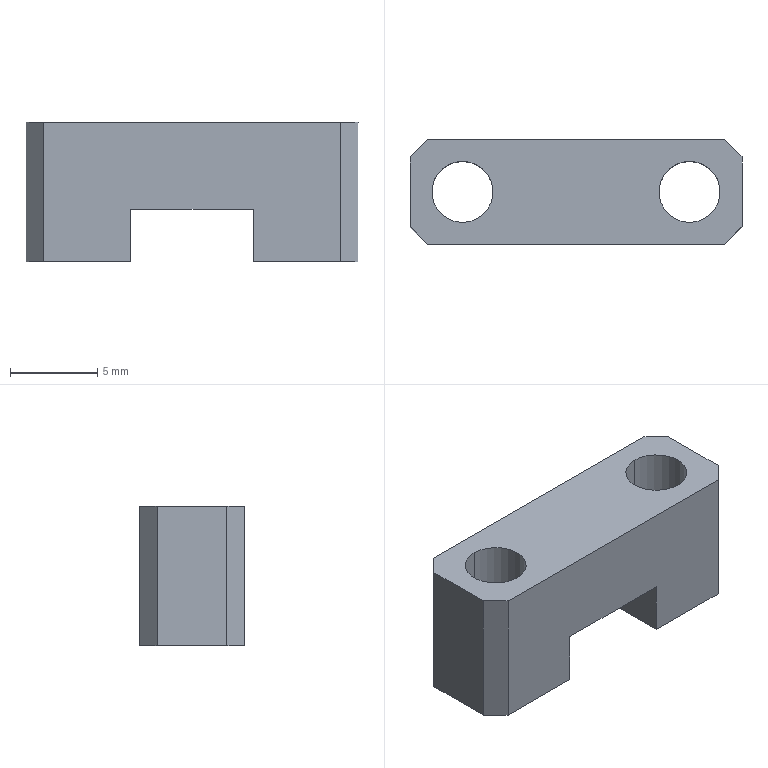Component | SolidWorks | F01AE00111-A5175-1 | 1 solid | 18 faces | box 19 x 6 x 8 mm | volume 616 mm3 | plane 14 | cylinder 4 | commonest cylinder face diameters 3.5 x4 | material 6061 Alloy
build123d program:
from build123d import *

# Parameters (mm, degrees)
BOSS_EXTRUDE1_DEPTH        = 3
F_3_5_3_5_DIAMETER_HOLE1_D = 3.5
CHAMFER1_SIZE              = 1


with BuildPart() as part:
    # Sketch1 → Boss-Extrude1 (new, symmetric)
    with BuildSketch(Plane.XY):
        Polygon((3.5, 0), (-3.5, 0), (-3.5, 3), (-9.5, 3), (-9.5, -5), (9.5, -5), (9.5, 3), (3.5, 3), align=None)
    extrude(amount=BOSS_EXTRUDE1_DEPTH, both=True)

    # 3.5 _3.5_ Diameter Hole1 (through all)
    with Locations(Plane(origin=(0, -5, 0), x_dir=(-1, 0, 0), z_dir=(0, -1, 0))):
        with Locations((-6.5, 0), (6.5, 0)):
            Hole(F_3_5_3_5_DIAMETER_HOLE1_D / 2)

    # Chamfer1
    chamfer1_edges = [part.edges().sort_by_distance(p)[0] for p in [
        (-9.5, -1, 3),
        (9.5, -1, 3),
        (9.5, -1, -3),
        (-9.5, -1, -3),
    ]]
    chamfer(chamfer1_edges, length=CHAMFER1_SIZE)


solid = part.part

# Placed as in the assembly
solid = solid.moved(Location((-63.681, -106.773, -304.179), (-90, 0, 0)))
STEP:
#1=CARTESIAN_POINT('',(-2.251,-4.135,-12.094));
#2=VERTEX_POINT('',#1);
#3=CARTESIAN_POINT('',(-2.251,-4.273,-12.094));
#4=VERTEX_POINT('',#3);
#5=CARTESIAN_POINT('',(-2.251,-4.204,-12.094));
#6=DIRECTION('',(0.,-0.,1.));
#7=DIRECTION('',(0.,-1.,0.));
#8=AXIS2_PLACEMENT_3D('',#5,#6,#7);
#9=CIRCLE('',#8,0.0689);
#10=EDGE_CURVE('',#2,#4,#9,.T.);
#11=ORIENTED_EDGE('',*,*,#10,.F.);
#12=CARTESIAN_POINT('',(-2.251,-4.135,-11.779));
#13=VERTEX_POINT('',#12);
#14=CARTESIAN_POINT('',(-2.251,-4.135,-11.779));
#15=DIRECTION('',(0.,-0.,1.));
#16=VECTOR('',#15,39.37);
#17=LINE('',#14,#16);
#18=EDGE_CURVE('',#2,#13,#17,.T.);
#19=ORIENTED_EDGE('',*,*,#18,.T.);
#20=CARTESIAN_POINT('',(-2.251,-4.273,-11.779));
#21=VERTEX_POINT('',#20);
#22=CARTESIAN_POINT('',(-2.251,-4.204,-11.779));
#23=DIRECTION('',(0.,-0.,1.));
#24=DIRECTION('',(0.,-1.,0.));
#25=AXIS2_PLACEMENT_3D('',#22,#23,#24);
#26=CIRCLE('',#25,0.0689);
#27=EDGE_CURVE('',#13,#21,#26,.T.);
#28=ORIENTED_EDGE('',*,*,#27,.T.);
#29=CARTESIAN_POINT('',(-2.251,-4.273,-11.779));
#30=DIRECTION('',(0.,-0.,1.));
#31=VECTOR('',#30,39.37);
#32=LINE('',#29,#31);
#33=EDGE_CURVE('',#4,#21,#32,.T.);
#34=ORIENTED_EDGE('',*,*,#33,.F.);
#35=EDGE_LOOP('',(#11,#19,#28,#34));
#36=FACE_OUTER_BOUND('',#35,.T.);
#37=CARTESIAN_POINT('',(-2.251,-4.204,-11.779));
#38=DIRECTION('',(0.,-0.,1.));
#39=DIRECTION('',(0.,-1.,0.));
#40=AXIS2_PLACEMENT_3D('',#37,#38,#39);
#41=CYLINDRICAL_SURFACE('',#40,0.0689);
#42=ADVANCED_FACE('',(#36),#41,.F.);
#43=CARTESIAN_POINT('',(-2.763,-4.135,-12.094));
#44=VERTEX_POINT('',#43);
#45=CARTESIAN_POINT('',(-2.763,-4.273,-12.094));
#46=VERTEX_POINT('',#45);
#47=CARTESIAN_POINT('',(-2.763,-4.204,-12.094));
#48=DIRECTION('',(0.,-0.,1.));
#49=DIRECTION('',(0.,-1.,0.));
#50=AXIS2_PLACEMENT_3D('',#47,#48,#49);
#51=CIRCLE('',#50,0.0689);
#52=EDGE_CURVE('',#44,#46,#51,.T.);
#53=ORIENTED_EDGE('',*,*,#52,.F.);
#54=CARTESIAN_POINT('',(-2.763,-4.135,-11.779));
#55=VERTEX_POINT('',#54);
#56=CARTESIAN_POINT('',(-2.763,-4.135,-11.779));
#57=DIRECTION('',(0.,-0.,1.));
#58=VECTOR('',#57,39.37);
#59=LINE('',#56,#58);
#60=EDGE_CURVE('',#44,#55,#59,.T.);
#61=ORIENTED_EDGE('',*,*,#60,.T.);
#62=CARTESIAN_POINT('',(-2.763,-4.273,-11.779));
#63=VERTEX_POINT('',#62);
#64=CARTESIAN_POINT('',(-2.763,-4.204,-11.779));
#65=DIRECTION('',(0.,-0.,1.));
#66=DIRECTION('',(0.,-1.,0.));
#67=AXIS2_PLACEMENT_3D('',#64,#65,#66);
#68=CIRCLE('',#67,0.0689);
#69=EDGE_CURVE('',#55,#63,#68,.T.);
#70=ORIENTED_EDGE('',*,*,#69,.T.);
#71=CARTESIAN_POINT('',(-2.763,-4.273,-11.779));
#72=DIRECTION('',(0.,-0.,1.));
#73=VECTOR('',#72,39.37);
#74=LINE('',#71,#73);
#75=EDGE_CURVE('',#46,#63,#74,.T.);
#76=ORIENTED_EDGE('',*,*,#75,.F.);
#77=EDGE_LOOP('',(#53,#61,#70,#76));
#78=FACE_OUTER_BOUND('',#77,.T.);
#79=CARTESIAN_POINT('',(-2.763,-4.204,-11.779));
#80=DIRECTION('',(0.,-0.,1.));
#81=DIRECTION('',(0.,-1.,0.));
#82=AXIS2_PLACEMENT_3D('',#79,#80,#81);
#83=CYLINDRICAL_SURFACE('',#82,0.0689);
#84=ADVANCED_FACE('',(#78),#83,.F.);
#85=CARTESIAN_POINT('',(-2.645,-4.322,-11.976));
#86=VERTEX_POINT('',#85);
#87=CARTESIAN_POINT('',(-2.645,-4.322,-12.094));
#88=VERTEX_POINT('',#87);
#89=CARTESIAN_POINT('',(-2.645,-4.322,-11.976));
#90=DIRECTION('',(-0.,0.,-1.));
#91=VECTOR('',#90,39.37);
#92=LINE('',#89,#91);
#93=EDGE_CURVE('',#86,#88,#92,.T.);
#94=ORIENTED_EDGE('',*,*,#93,.T.);
#95=CARTESIAN_POINT('',(-2.645,-4.086,-12.094));
#96=VERTEX_POINT('',#95);
#97=CARTESIAN_POINT('',(-2.645,-4.086,-12.094));
#98=DIRECTION('',(-0.,-1.,-0.));
#99=VECTOR('',#98,39.37);
#100=LINE('',#97,#99);
#101=EDGE_CURVE('',#96,#88,#100,.T.);
#102=ORIENTED_EDGE('',*,*,#101,.F.);
#103=CARTESIAN_POINT('',(-2.645,-4.086,-11.976));
#104=VERTEX_POINT('',#103);
#105=CARTESIAN_POINT('',(-2.645,-4.086,-11.976));
#106=DIRECTION('',(-0.,0.,-1.));
#107=VECTOR('',#106,39.37);
#108=LINE('',#105,#107);
#109=EDGE_CURVE('',#104,#96,#108,.T.);
#110=ORIENTED_EDGE('',*,*,#109,.F.);
#111=CARTESIAN_POINT('',(-2.645,-4.086,-11.976));
#112=DIRECTION('',(-0.,-1.,-0.));
#113=VECTOR('',#112,39.37);
#114=LINE('',#111,#113);
#115=EDGE_CURVE('',#104,#86,#114,.T.);
#116=ORIENTED_EDGE('',*,*,#115,.T.);
#117=EDGE_LOOP('',(#94,#102,#110,#116));
#118=FACE_OUTER_BOUND('',#117,.T.);
#119=CARTESIAN_POINT('',(-2.645,-4.086,-11.976));
#120=DIRECTION('',(-1.,0.,0.));
#121=DIRECTION('',(0.,1.,0.));
#122=AXIS2_PLACEMENT_3D('',#119,#120,#121);
#123=PLANE('',#122);
#124=ADVANCED_FACE('',(#118),#123,.F.);
#125=CARTESIAN_POINT('',(-2.763,-4.204,-12.094));
#126=DIRECTION('',(0.,-0.,1.));
#127=DIRECTION('',(0.,-1.,0.));
#128=AXIS2_PLACEMENT_3D('',#125,#126,#127);
#129=CIRCLE('',#128,0.0689);
#130=EDGE_CURVE('',#46,#44,#129,.T.);
#131=ORIENTED_EDGE('',*,*,#130,.T.);
#132=ORIENTED_EDGE('',*,*,#52,.T.);
#133=EDGE_LOOP('',(#131,#132));
#134=FACE_BOUND('',#133,.T.);
#135=CARTESIAN_POINT('',(-2.842,-4.322,-12.094));
#136=VERTEX_POINT('',#135);
#137=CARTESIAN_POINT('',(-2.645,-4.322,-12.094));
#138=DIRECTION('',(-1.,0.,0.));
#139=VECTOR('',#138,39.37);
#140=LINE('',#137,#139);
#141=EDGE_CURVE('',#88,#136,#140,.T.);
#142=ORIENTED_EDGE('',*,*,#141,.T.);
#143=CARTESIAN_POINT('',(-2.881,-4.282,-12.094));
#144=VERTEX_POINT('',#143);
#145=CARTESIAN_POINT('',(-2.881,-4.282,-12.094));
#146=DIRECTION('',(-0.7071,0.7071,0.));
#147=VECTOR('',#146,39.37);
#148=LINE('',#145,#147);
#149=EDGE_CURVE('',#136,#144,#148,.T.);
#150=ORIENTED_EDGE('',*,*,#149,.T.);
#151=CARTESIAN_POINT('',(-2.881,-4.125,-12.094));
#152=VERTEX_POINT('',#151);
#153=CARTESIAN_POINT('',(-2.881,-4.086,-12.094));
#154=DIRECTION('',(-0.,-1.,-0.));
#155=VECTOR('',#154,39.37);
#156=LINE('',#153,#155);
#157=EDGE_CURVE('',#152,#144,#156,.T.);
#158=ORIENTED_EDGE('',*,*,#157,.F.);
#159=CARTESIAN_POINT('',(-2.842,-4.086,-12.094));
#160=VERTEX_POINT('',#159);
#161=CARTESIAN_POINT('',(-2.842,-4.086,-12.094));
#162=DIRECTION('',(0.7071,0.7071,-0.));
#163=VECTOR('',#162,39.37);
#164=LINE('',#161,#163);
#165=EDGE_CURVE('',#152,#160,#164,.T.);
#166=ORIENTED_EDGE('',*,*,#165,.T.);
#167=CARTESIAN_POINT('',(-2.645,-4.086,-12.094));
#168=DIRECTION('',(-1.,0.,0.));
#169=VECTOR('',#168,39.37);
#170=LINE('',#167,#169);
#171=EDGE_CURVE('',#96,#160,#170,.T.);
#172=ORIENTED_EDGE('',*,*,#171,.F.);
#173=ORIENTED_EDGE('',*,*,#101,.T.);
#174=EDGE_LOOP('',(#142,#150,#158,#166,#172,#173));
#175=FACE_OUTER_BOUND('',#174,.T.);
#176=CARTESIAN_POINT('',(-2.645,-4.086,-12.094));
#177=DIRECTION('',(0.,-0.,1.));
#178=DIRECTION('',(-0.,-1.,-0.));
#179=AXIS2_PLACEMENT_3D('',#176,#177,#178);
#180=PLANE('',#179);
#181=ADVANCED_FACE('',(#134,#175),#180,.F.);
#182=ORIENTED_EDGE('',*,*,#157,.T.);
#183=CARTESIAN_POINT('',(-2.881,-4.282,-11.779));
#184=VERTEX_POINT('',#183);
#185=CARTESIAN_POINT('',(-2.881,-4.282,-12.094));
#186=DIRECTION('',(0.,-0.,1.));
#187=VECTOR('',#186,39.37);
#188=LINE('',#185,#187);
#189=EDGE_CURVE('',#144,#184,#188,.T.);
#190=ORIENTED_EDGE('',*,*,#189,.T.);
#191=CARTESIAN_POINT('',(-2.881,-4.125,-11.779));
#192=VERTEX_POINT('',#191);
#193=CARTESIAN_POINT('',(-2.881,-4.086,-11.779));
#194=DIRECTION('',(-0.,-1.,-0.));
#195=VECTOR('',#194,39.37);
#196=LINE('',#193,#195);
#197=EDGE_CURVE('',#192,#184,#196,.T.);
#198=ORIENTED_EDGE('',*,*,#197,.F.);
#199=CARTESIAN_POINT('',(-2.881,-4.125,-12.094));
#200=DIRECTION('',(-0.,0.,-1.));
#201=VECTOR('',#200,39.37);
#202=LINE('',#199,#201);
#203=EDGE_CURVE('',#192,#152,#202,.T.);
#204=ORIENTED_EDGE('',*,*,#203,.T.);
#205=EDGE_LOOP('',(#182,#190,#198,#204));
#206=FACE_OUTER_BOUND('',#205,.T.);
#207=CARTESIAN_POINT('',(-2.881,-4.086,-12.094));
#208=DIRECTION('',(1.,-0.,-0.));
#209=DIRECTION('',(-0.,0.,-1.));
#210=AXIS2_PLACEMENT_3D('',#207,#208,#209);
#211=PLANE('',#210);
#212=ADVANCED_FACE('',(#206),#211,.F.);
#213=CARTESIAN_POINT('',(-2.251,-4.204,-11.779));
#214=DIRECTION('',(0.,-0.,1.));
#215=DIRECTION('',(0.,-1.,0.));
#216=AXIS2_PLACEMENT_3D('',#213,#214,#215);
#217=CIRCLE('',#216,0.0689);
#218=EDGE_CURVE('',#21,#13,#217,.T.);
#219=ORIENTED_EDGE('',*,*,#218,.F.);
#220=ORIENTED_EDGE('',*,*,#27,.F.);
#221=EDGE_LOOP('',(#219,#220));
#222=FACE_BOUND('',#221,.T.);
#223=CARTESIAN_POINT('',(-2.763,-4.204,-11.779));
#224=DIRECTION('',(0.,-0.,1.));
#225=DIRECTION('',(0.,-1.,0.));
#226=AXIS2_PLACEMENT_3D('',#223,#224,#225);
#227=CIRCLE('',#226,0.0689);
#228=EDGE_CURVE('',#63,#55,#227,.T.);
#229=ORIENTED_EDGE('',*,*,#228,.F.);
#230=ORIENTED_EDGE('',*,*,#69,.F.);
#231=EDGE_LOOP('',(#229,#230));
#232=FACE_BOUND('',#231,.T.);
#233=CARTESIAN_POINT('',(-2.842,-4.322,-11.779));
#234=VERTEX_POINT('',#233);
#235=CARTESIAN_POINT('',(-2.172,-4.322,-11.779));
#236=VERTEX_POINT('',#235);
#237=CARTESIAN_POINT('',(-2.881,-4.322,-11.779));
#238=DIRECTION('',(1.,-0.,-0.));
#239=VECTOR('',#238,39.37);
#240=LINE('',#237,#239);
#241=EDGE_CURVE('',#234,#236,#240,.T.);
#242=ORIENTED_EDGE('',*,*,#241,.T.);
#243=CARTESIAN_POINT('',(-2.133,-4.282,-11.779));
#244=VERTEX_POINT('',#243);
#245=CARTESIAN_POINT('',(-2.133,-4.282,-11.779));
#246=DIRECTION('',(0.7071,0.7071,-0.));
#247=VECTOR('',#246,39.37);
#248=LINE('',#245,#247);
#249=EDGE_CURVE('',#236,#244,#248,.T.);
#250=ORIENTED_EDGE('',*,*,#249,.T.);
#251=CARTESIAN_POINT('',(-2.133,-4.125,-11.779));
#252=VERTEX_POINT('',#251);
#253=CARTESIAN_POINT('',(-2.133,-4.086,-11.779));
#254=DIRECTION('',(-0.,-1.,-0.));
#255=VECTOR('',#254,39.37);
#256=LINE('',#253,#255);
#257=EDGE_CURVE('',#252,#244,#256,.T.);
#258=ORIENTED_EDGE('',*,*,#257,.F.);
#259=CARTESIAN_POINT('',(-2.172,-4.086,-11.779));
#260=VERTEX_POINT('',#259);
#261=CARTESIAN_POINT('',(-2.172,-4.086,-11.779));
#262=DIRECTION('',(-0.7071,0.7071,0.));
#263=VECTOR('',#262,39.37);
#264=LINE('',#261,#263);
#265=EDGE_CURVE('',#252,#260,#264,.T.);
#266=ORIENTED_EDGE('',*,*,#265,.T.);
#267=CARTESIAN_POINT('',(-2.842,-4.086,-11.779));
#268=VERTEX_POINT('',#267);
#269=CARTESIAN_POINT('',(-2.881,-4.086,-11.779));
#270=DIRECTION('',(1.,-0.,-0.));
#271=VECTOR('',#270,39.37);
#272=LINE('',#269,#271);
#273=EDGE_CURVE('',#268,#260,#272,.T.);
#274=ORIENTED_EDGE('',*,*,#273,.F.);
#275=CARTESIAN_POINT('',(-2.842,-4.086,-11.779));
#276=DIRECTION('',(-0.7071,-0.7071,0.));
#277=VECTOR('',#276,39.37);
#278=LINE('',#275,#277);
#279=EDGE_CURVE('',#268,#192,#278,.T.);
#280=ORIENTED_EDGE('',*,*,#279,.T.);
#281=ORIENTED_EDGE('',*,*,#197,.T.);
#282=CARTESIAN_POINT('',(-2.881,-4.282,-11.779));
#283=DIRECTION('',(0.7071,-0.7071,-0.));
#284=VECTOR('',#283,39.37);
#285=LINE('',#282,#284);
#286=EDGE_CURVE('',#184,#234,#285,.T.);
#287=ORIENTED_EDGE('',*,*,#286,.T.);
#288=EDGE_LOOP('',(#242,#250,#258,#266,#274,#280,#281,#287));
#289=FACE_OUTER_BOUND('',#288,.T.);
#290=CARTESIAN_POINT('',(-2.881,-4.086,-11.779));
#291=DIRECTION('',(-0.,0.,-1.));
#292=DIRECTION('',(-1.,0.,0.));
#293=AXIS2_PLACEMENT_3D('',#290,#291,#292);
#294=PLANE('',#293);
#295=ADVANCED_FACE('',(#222,#232,#289),#294,.F.);
#296=ORIENTED_EDGE('',*,*,#257,.T.);
#297=CARTESIAN_POINT('',(-2.133,-4.282,-12.094));
#298=VERTEX_POINT('',#297);
#299=CARTESIAN_POINT('',(-2.133,-4.282,-12.094));
#300=DIRECTION('',(-0.,0.,-1.));
#301=VECTOR('',#300,39.37);
#302=LINE('',#299,#301);
#303=EDGE_CURVE('',#244,#298,#302,.T.);
#304=ORIENTED_EDGE('',*,*,#303,.T.);
#305=CARTESIAN_POINT('',(-2.133,-4.125,-12.094));
#306=VERTEX_POINT('',#305);
#307=CARTESIAN_POINT('',(-2.133,-4.086,-12.094));
#308=DIRECTION('',(-0.,-1.,-0.));
#309=VECTOR('',#308,39.37);
#310=LINE('',#307,#309);
#311=EDGE_CURVE('',#306,#298,#310,.T.);
#312=ORIENTED_EDGE('',*,*,#311,.F.);
#313=CARTESIAN_POINT('',(-2.133,-4.125,-11.779));
#314=DIRECTION('',(0.,-0.,1.));
#315=VECTOR('',#314,39.37);
#316=LINE('',#313,#315);
#317=EDGE_CURVE('',#306,#252,#316,.T.);
#318=ORIENTED_EDGE('',*,*,#317,.T.);
#319=EDGE_LOOP('',(#296,#304,#312,#318));
#320=FACE_OUTER_BOUND('',#319,.T.);
#321=CARTESIAN_POINT('',(-2.133,-4.086,-12.094));
#322=DIRECTION('',(-1.,0.,0.));
#323=DIRECTION('',(0.,-0.,1.));
#324=AXIS2_PLACEMENT_3D('',#321,#322,#323);
#325=PLANE('',#324);
#326=ADVANCED_FACE('',(#320),#325,.F.);
#327=CARTESIAN_POINT('',(-2.251,-4.204,-12.094));
#328=DIRECTION('',(0.,-0.,1.));
#329=DIRECTION('',(0.,-1.,0.));
#330=AXIS2_PLACEMENT_3D('',#327,#328,#329);
#331=CIRCLE('',#330,0.0689);
#332=EDGE_CURVE('',#4,#2,#331,.T.);
#333=ORIENTED_EDGE('',*,*,#332,.T.);
#334=ORIENTED_EDGE('',*,*,#10,.T.);
#335=EDGE_LOOP('',(#333,#334));
#336=FACE_BOUND('',#335,.T.);
#337=ORIENTED_EDGE('',*,*,#311,.T.);
#338=CARTESIAN_POINT('',(-2.172,-4.322,-12.094));
#339=VERTEX_POINT('',#338);
#340=CARTESIAN_POINT('',(-2.133,-4.282,-12.094));
#341=DIRECTION('',(-0.7071,-0.7071,0.));
#342=VECTOR('',#341,39.37);
#343=LINE('',#340,#342);
#344=EDGE_CURVE('',#298,#339,#343,.T.);
#345=ORIENTED_EDGE('',*,*,#344,.T.);
#346=CARTESIAN_POINT('',(-2.369,-4.322,-12.094));
#347=VERTEX_POINT('',#346);
#348=CARTESIAN_POINT('',(-2.369,-4.322,-12.094));
#349=DIRECTION('',(-1.,0.,0.));
#350=VECTOR('',#349,39.37);
#351=LINE('',#348,#350);
#352=EDGE_CURVE('',#339,#347,#351,.T.);
#353=ORIENTED_EDGE('',*,*,#352,.T.);
#354=CARTESIAN_POINT('',(-2.369,-4.086,-12.094));
#355=VERTEX_POINT('',#354);
#356=CARTESIAN_POINT('',(-2.369,-4.086,-12.094));
#357=DIRECTION('',(-0.,-1.,-0.));
#358=VECTOR('',#357,39.37);
#359=LINE('',#356,#358);
#360=EDGE_CURVE('',#355,#347,#359,.T.);
#361=ORIENTED_EDGE('',*,*,#360,.F.);
#362=CARTESIAN_POINT('',(-2.172,-4.086,-12.094));
#363=VERTEX_POINT('',#362);
#364=CARTESIAN_POINT('',(-2.369,-4.086,-12.094));
#365=DIRECTION('',(-1.,0.,0.));
#366=VECTOR('',#365,39.37);
#367=LINE('',#364,#366);
#368=EDGE_CURVE('',#363,#355,#367,.T.);
#369=ORIENTED_EDGE('',*,*,#368,.F.);
#370=CARTESIAN_POINT('',(-2.172,-4.086,-12.094));
#371=DIRECTION('',(0.7071,-0.7071,-0.));
#372=VECTOR('',#371,39.37);
#373=LINE('',#370,#372);
#374=EDGE_CURVE('',#363,#306,#373,.T.);
#375=ORIENTED_EDGE('',*,*,#374,.T.);
#376=EDGE_LOOP('',(#337,#345,#353,#361,#369,#375));
#377=FACE_OUTER_BOUND('',#376,.T.);
#378=CARTESIAN_POINT('',(-2.369,-4.086,-12.094));
#379=DIRECTION('',(0.,-0.,1.));
#380=DIRECTION('',(1.,-0.,-0.));
#381=AXIS2_PLACEMENT_3D('',#378,#379,#380);
#382=PLANE('',#381);
#383=ADVANCED_FACE('',(#336,#377),#382,.F.);
#384=CARTESIAN_POINT('',(-2.369,-4.322,-11.976));
#385=VERTEX_POINT('',#384);
#386=CARTESIAN_POINT('',(-2.369,-4.322,-11.976));
#387=DIRECTION('',(0.,-0.,1.));
#388=VECTOR('',#387,39.37);
#389=LINE('',#386,#388);
#390=EDGE_CURVE('',#347,#385,#389,.T.);
#391=ORIENTED_EDGE('',*,*,#390,.T.);
#392=CARTESIAN_POINT('',(-2.369,-4.086,-11.976));
#393=VERTEX_POINT('',#392);
#394=CARTESIAN_POINT('',(-2.369,-4.086,-11.976));
#395=DIRECTION('',(-0.,-1.,-0.));
#396=VECTOR('',#395,39.37);
#397=LINE('',#394,#396);
#398=EDGE_CURVE('',#393,#385,#397,.T.);
#399=ORIENTED_EDGE('',*,*,#398,.F.);
#400=CARTESIAN_POINT('',(-2.369,-4.086,-11.976));
#401=DIRECTION('',(0.,-0.,1.));
#402=VECTOR('',#401,39.37);
#403=LINE('',#400,#402);
#404=EDGE_CURVE('',#355,#393,#403,.T.);
#405=ORIENTED_EDGE('',*,*,#404,.F.);
#406=ORIENTED_EDGE('',*,*,#360,.T.);
#407=EDGE_LOOP('',(#391,#399,#405,#406));
#408=FACE_OUTER_BOUND('',#407,.T.);
#409=CARTESIAN_POINT('',(-2.369,-4.086,-11.976));
#410=DIRECTION('',(1.,-0.,-0.));
#411=DIRECTION('',(-0.,0.,-1.));
#412=AXIS2_PLACEMENT_3D('',#409,#410,#411);
#413=PLANE('',#412);
#414=ADVANCED_FACE('',(#408),#413,.F.);
#415=CARTESIAN_POINT('',(-2.369,-4.322,-11.976));
#416=DIRECTION('',(-1.,0.,0.));
#417=VECTOR('',#416,39.37);
#418=LINE('',#415,#417);
#419=EDGE_CURVE('',#385,#86,#418,.T.);
#420=ORIENTED_EDGE('',*,*,#419,.T.);
#421=ORIENTED_EDGE('',*,*,#115,.F.);
#422=CARTESIAN_POINT('',(-2.369,-4.086,-11.976));
#423=DIRECTION('',(-1.,0.,0.));
#424=VECTOR('',#423,39.37);
#425=LINE('',#422,#424);
#426=EDGE_CURVE('',#393,#104,#425,.T.);
#427=ORIENTED_EDGE('',*,*,#426,.F.);
#428=ORIENTED_EDGE('',*,*,#398,.T.);
#429=EDGE_LOOP('',(#420,#421,#427,#428));
#430=FACE_OUTER_BOUND('',#429,.T.);
#431=CARTESIAN_POINT('',(-2.369,-4.086,-11.976));
#432=DIRECTION('',(0.,-0.,1.));
#433=DIRECTION('',(1.,-0.,-0.));
#434=AXIS2_PLACEMENT_3D('',#431,#432,#433);
#435=PLANE('',#434);
#436=ADVANCED_FACE('',(#430),#435,.F.);
#437=ORIENTED_EDGE('',*,*,#273,.T.);
#438=CARTESIAN_POINT('',(-2.172,-4.086,-12.094));
#439=DIRECTION('',(-0.,0.,-1.));
#440=VECTOR('',#439,39.37);
#441=LINE('',#438,#440);
#442=EDGE_CURVE('',#260,#363,#441,.T.);
#443=ORIENTED_EDGE('',*,*,#442,.T.);
#444=ORIENTED_EDGE('',*,*,#368,.T.);
#445=ORIENTED_EDGE('',*,*,#404,.T.);
#446=ORIENTED_EDGE('',*,*,#426,.T.);
#447=ORIENTED_EDGE('',*,*,#109,.T.);
#448=ORIENTED_EDGE('',*,*,#171,.T.);
#449=CARTESIAN_POINT('',(-2.842,-4.086,-11.779));
#450=DIRECTION('',(0.,-0.,1.));
#451=VECTOR('',#450,39.37);
#452=LINE('',#449,#451);
#453=EDGE_CURVE('',#160,#268,#452,.T.);
#454=ORIENTED_EDGE('',*,*,#453,.T.);
#455=EDGE_LOOP('',(#437,#443,#444,#445,#446,#447,#448,#454));
#456=FACE_OUTER_BOUND('',#455,.T.);
#457=CARTESIAN_POINT('',(-2.507,-4.086,-11.976));
#458=DIRECTION('',(0.,1.,0.));
#459=DIRECTION('',(1.,-0.,-0.));
#460=AXIS2_PLACEMENT_3D('',#457,#458,#459);
#461=PLANE('',#460);
#462=ADVANCED_FACE('',(#456),#461,.T.);
#463=ORIENTED_EDGE('',*,*,#352,.F.);
#464=CARTESIAN_POINT('',(-2.172,-4.322,-11.976));
#465=DIRECTION('',(0.,-0.,1.));
#466=VECTOR('',#465,39.37);
#467=LINE('',#464,#466);
#468=EDGE_CURVE('',#339,#236,#467,.T.);
#469=ORIENTED_EDGE('',*,*,#468,.T.);
#470=ORIENTED_EDGE('',*,*,#241,.F.);
#471=CARTESIAN_POINT('',(-2.842,-4.322,-11.976));
#472=DIRECTION('',(-0.,0.,-1.));
#473=VECTOR('',#472,39.37);
#474=LINE('',#471,#473);
#475=EDGE_CURVE('',#234,#136,#474,.T.);
#476=ORIENTED_EDGE('',*,*,#475,.T.);
#477=ORIENTED_EDGE('',*,*,#141,.F.);
#478=ORIENTED_EDGE('',*,*,#93,.F.);
#479=ORIENTED_EDGE('',*,*,#419,.F.);
#480=ORIENTED_EDGE('',*,*,#390,.F.);
#481=EDGE_LOOP('',(#463,#469,#470,#476,#477,#478,#479,#480));
#482=FACE_OUTER_BOUND('',#481,.T.);
#483=CARTESIAN_POINT('',(-2.507,-4.322,-11.976));
#484=DIRECTION('',(0.,1.,0.));
#485=DIRECTION('',(1.,-0.,-0.));
#486=AXIS2_PLACEMENT_3D('',#483,#484,#485);
#487=PLANE('',#486);
#488=ADVANCED_FACE('',(#482),#487,.F.);
#489=ORIENTED_EDGE('',*,*,#60,.F.);
#490=ORIENTED_EDGE('',*,*,#130,.F.);
#491=ORIENTED_EDGE('',*,*,#75,.T.);
#492=ORIENTED_EDGE('',*,*,#228,.T.);
#493=EDGE_LOOP('',(#489,#490,#491,#492));
#494=FACE_OUTER_BOUND('',#493,.T.);
#495=CARTESIAN_POINT('',(-2.763,-4.204,-11.779));
#496=DIRECTION('',(0.,-0.,1.));
#497=DIRECTION('',(0.,-1.,0.));
#498=AXIS2_PLACEMENT_3D('',#495,#496,#497);
#499=CYLINDRICAL_SURFACE('',#498,0.0689);
#500=ADVANCED_FACE('',(#494),#499,.F.);
#501=ORIENTED_EDGE('',*,*,#18,.F.);
#502=ORIENTED_EDGE('',*,*,#332,.F.);
#503=ORIENTED_EDGE('',*,*,#33,.T.);
#504=ORIENTED_EDGE('',*,*,#218,.T.);
#505=EDGE_LOOP('',(#501,#502,#503,#504));
#506=FACE_OUTER_BOUND('',#505,.T.);
#507=CARTESIAN_POINT('',(-2.251,-4.204,-11.779));
#508=DIRECTION('',(0.,-0.,1.));
#509=DIRECTION('',(0.,-1.,0.));
#510=AXIS2_PLACEMENT_3D('',#507,#508,#509);
#511=CYLINDRICAL_SURFACE('',#510,0.0689);
#512=ADVANCED_FACE('',(#506),#511,.F.);
#513=ORIENTED_EDGE('',*,*,#249,.F.);
#514=ORIENTED_EDGE('',*,*,#468,.F.);
#515=ORIENTED_EDGE('',*,*,#344,.F.);
#516=ORIENTED_EDGE('',*,*,#303,.F.);
#517=EDGE_LOOP('',(#513,#514,#515,#516));
#518=FACE_OUTER_BOUND('',#517,.T.);
#519=CARTESIAN_POINT('',(-2.133,-4.282,-12.094));
#520=DIRECTION('',(-0.7071,0.7071,0.));
#521=DIRECTION('',(-0.,0.,-1.));
#522=AXIS2_PLACEMENT_3D('',#519,#520,#521);
#523=PLANE('',#522);
#524=ADVANCED_FACE('',(#518),#523,.F.);
#525=ORIENTED_EDGE('',*,*,#265,.F.);
#526=ORIENTED_EDGE('',*,*,#317,.F.);
#527=ORIENTED_EDGE('',*,*,#374,.F.);
#528=ORIENTED_EDGE('',*,*,#442,.F.);
#529=EDGE_LOOP('',(#525,#526,#527,#528));
#530=FACE_OUTER_BOUND('',#529,.T.);
#531=CARTESIAN_POINT('',(-2.172,-4.086,-11.976));
#532=DIRECTION('',(0.7071,0.7071,-0.));
#533=DIRECTION('',(0.,-0.,1.));
#534=AXIS2_PLACEMENT_3D('',#531,#532,#533);
#535=PLANE('',#534);
#536=ADVANCED_FACE('',(#530),#535,.T.);
#537=ORIENTED_EDGE('',*,*,#149,.F.);
#538=ORIENTED_EDGE('',*,*,#475,.F.);
#539=ORIENTED_EDGE('',*,*,#286,.F.);
#540=ORIENTED_EDGE('',*,*,#189,.F.);
#541=EDGE_LOOP('',(#537,#538,#539,#540));
#542=FACE_OUTER_BOUND('',#541,.T.);
#543=CARTESIAN_POINT('',(-2.881,-4.282,-12.094));
#544=DIRECTION('',(0.7071,0.7071,-0.));
#545=DIRECTION('',(0.,-0.,1.));
#546=AXIS2_PLACEMENT_3D('',#543,#544,#545);
#547=PLANE('',#546);
#548=ADVANCED_FACE('',(#542),#547,.F.);
#549=ORIENTED_EDGE('',*,*,#165,.F.);
#550=ORIENTED_EDGE('',*,*,#203,.F.);
#551=ORIENTED_EDGE('',*,*,#279,.F.);
#552=ORIENTED_EDGE('',*,*,#453,.F.);
#553=EDGE_LOOP('',(#549,#550,#551,#552));
#554=FACE_OUTER_BOUND('',#553,.T.);
#555=CARTESIAN_POINT('',(-2.842,-4.086,-11.976));
#556=DIRECTION('',(-0.7071,0.7071,0.));
#557=DIRECTION('',(-0.,0.,-1.));
#558=AXIS2_PLACEMENT_3D('',#555,#556,#557);
#559=PLANE('',#558);
#560=ADVANCED_FACE('',(#554),#559,.T.);
#561=CLOSED_SHELL('',(#42,#84,#124,#181,#212,#295,#326,#383,#414,#436,#462,#488,#500,#512,#524,#536,#548,#560));
#562=MANIFOLD_SOLID_BREP('',#561);
#563=CARTESIAN_POINT('',(0.,0.,0.));
#564=DIRECTION('',(0.,0.,1.));
#565=DIRECTION('',(1.,0.,0.));
#566=AXIS2_PLACEMENT_3D('',#563,#564,#565);
#567=(LENGTH_UNIT()NAMED_UNIT(*)SI_UNIT($,.METRE.));
#568=LENGTH_MEASURE_WITH_UNIT(LENGTH_MEASURE(0.0254),#567);
#569=DIMENSIONAL_EXPONENTS(1.,0.,0.,0.,0.,0.,0.);
#570=(CONVERSION_BASED_UNIT('',#568)LENGTH_UNIT()NAMED_UNIT(#569));
#571=UNCERTAINTY_MEASURE_WITH_UNIT(LENGTH_MEASURE(0.00001),#570,'','');
#572=(NAMED_UNIT(*)PLANE_ANGLE_UNIT()SI_UNIT($,.RADIAN.));
#573=(NAMED_UNIT(*)SI_UNIT($,.STERADIAN.)SOLID_ANGLE_UNIT());
#574=(GEOMETRIC_REPRESENTATION_CONTEXT(3)GLOBAL_UNCERTAINTY_ASSIGNED_CONTEXT((#571))GLOBAL_UNIT_ASSIGNED_CONTEXT((#570,#572,#573))REPRESENTATION_CONTEXT('',''));
#575=ADVANCED_BREP_SHAPE_REPRESENTATION('',(#562,#566),#574);
#576=COLOUR_RGB('',0.7922,0.8196,0.9333);
#577=FILL_AREA_STYLE_COLOUR('',#576);
#578=FILL_AREA_STYLE('',(#577));
#579=SURFACE_STYLE_FILL_AREA(#578);
#580=SURFACE_SIDE_STYLE('',(#579));
#581=SURFACE_STYLE_USAGE(.BOTH.,#580);
#582=PRESENTATION_STYLE_ASSIGNMENT((#581));
#583=STYLED_ITEM('',(#582),#562);
#584=(LENGTH_UNIT()NAMED_UNIT(*)SI_UNIT($,.METRE.));
#585=LENGTH_MEASURE_WITH_UNIT(LENGTH_MEASURE(0.0254),#584);
#586=DIMENSIONAL_EXPONENTS(1.,0.,0.,0.,0.,0.,0.);
#587=(CONVERSION_BASED_UNIT('',#585)LENGTH_UNIT()NAMED_UNIT(#586));
#588=UNCERTAINTY_MEASURE_WITH_UNIT(LENGTH_MEASURE(0.00001),#587,'','');
#589=(NAMED_UNIT(*)PLANE_ANGLE_UNIT()SI_UNIT($,.RADIAN.));
#590=(NAMED_UNIT(*)SI_UNIT($,.STERADIAN.)SOLID_ANGLE_UNIT());
#591=(GEOMETRIC_REPRESENTATION_CONTEXT(3)GLOBAL_UNCERTAINTY_ASSIGNED_CONTEXT((#588))GLOBAL_UNIT_ASSIGNED_CONTEXT((#587,#589,#590))REPRESENTATION_CONTEXT('',''));
#592=MECHANICAL_DESIGN_GEOMETRIC_PRESENTATION_REPRESENTATION('',(#583),#591);
#593=PRESENTATION_LAYER_ASSIGNMENT('','',(#583));